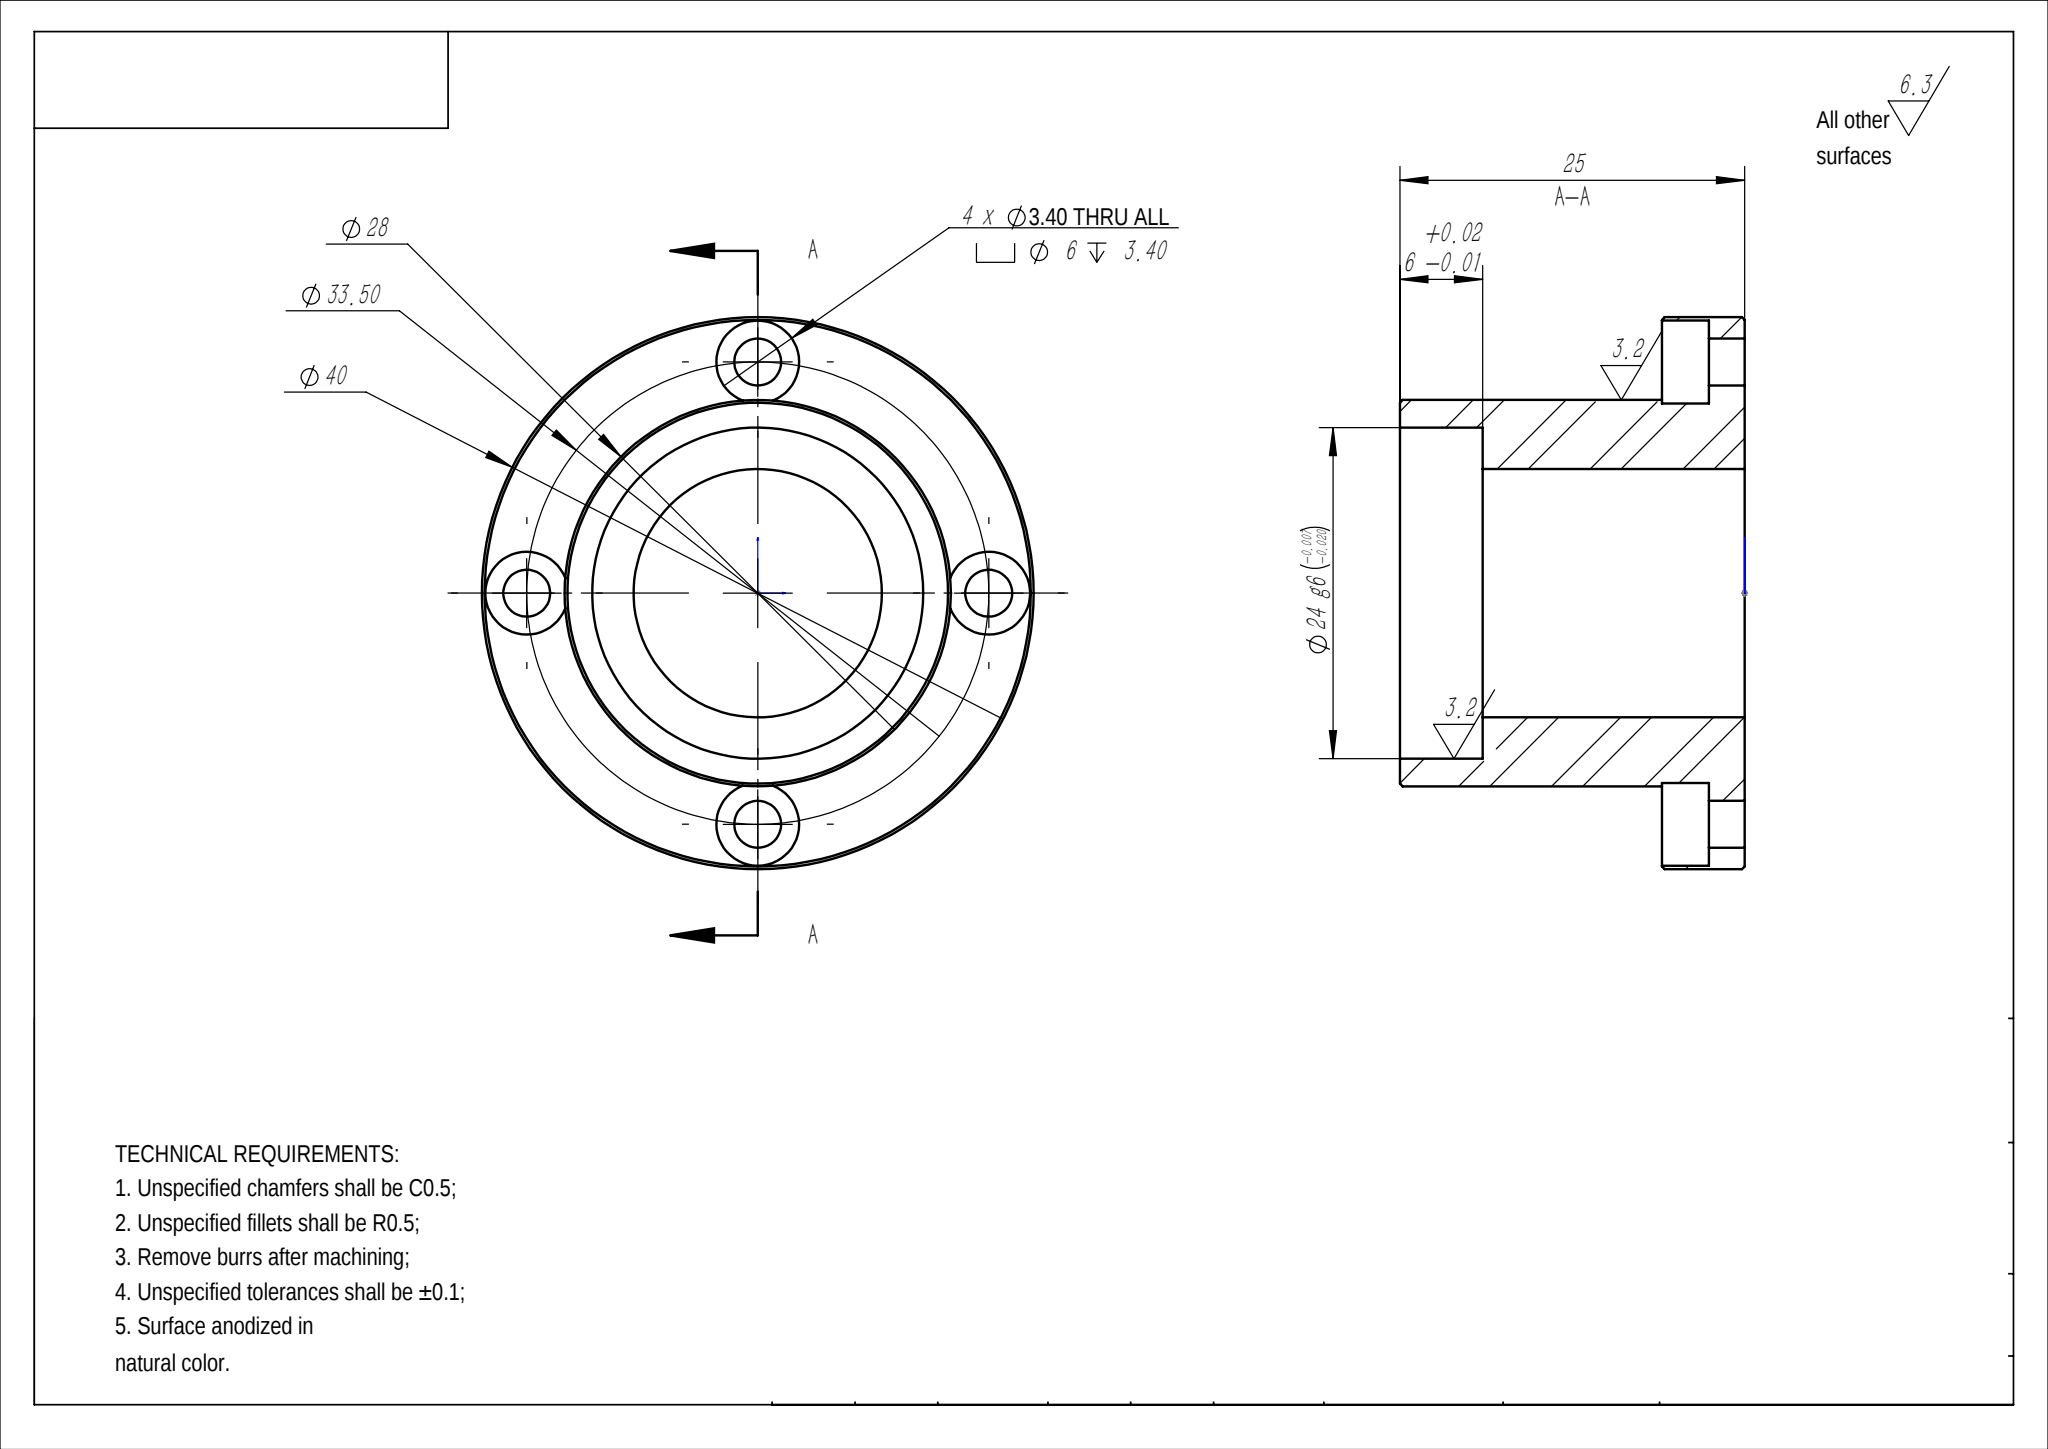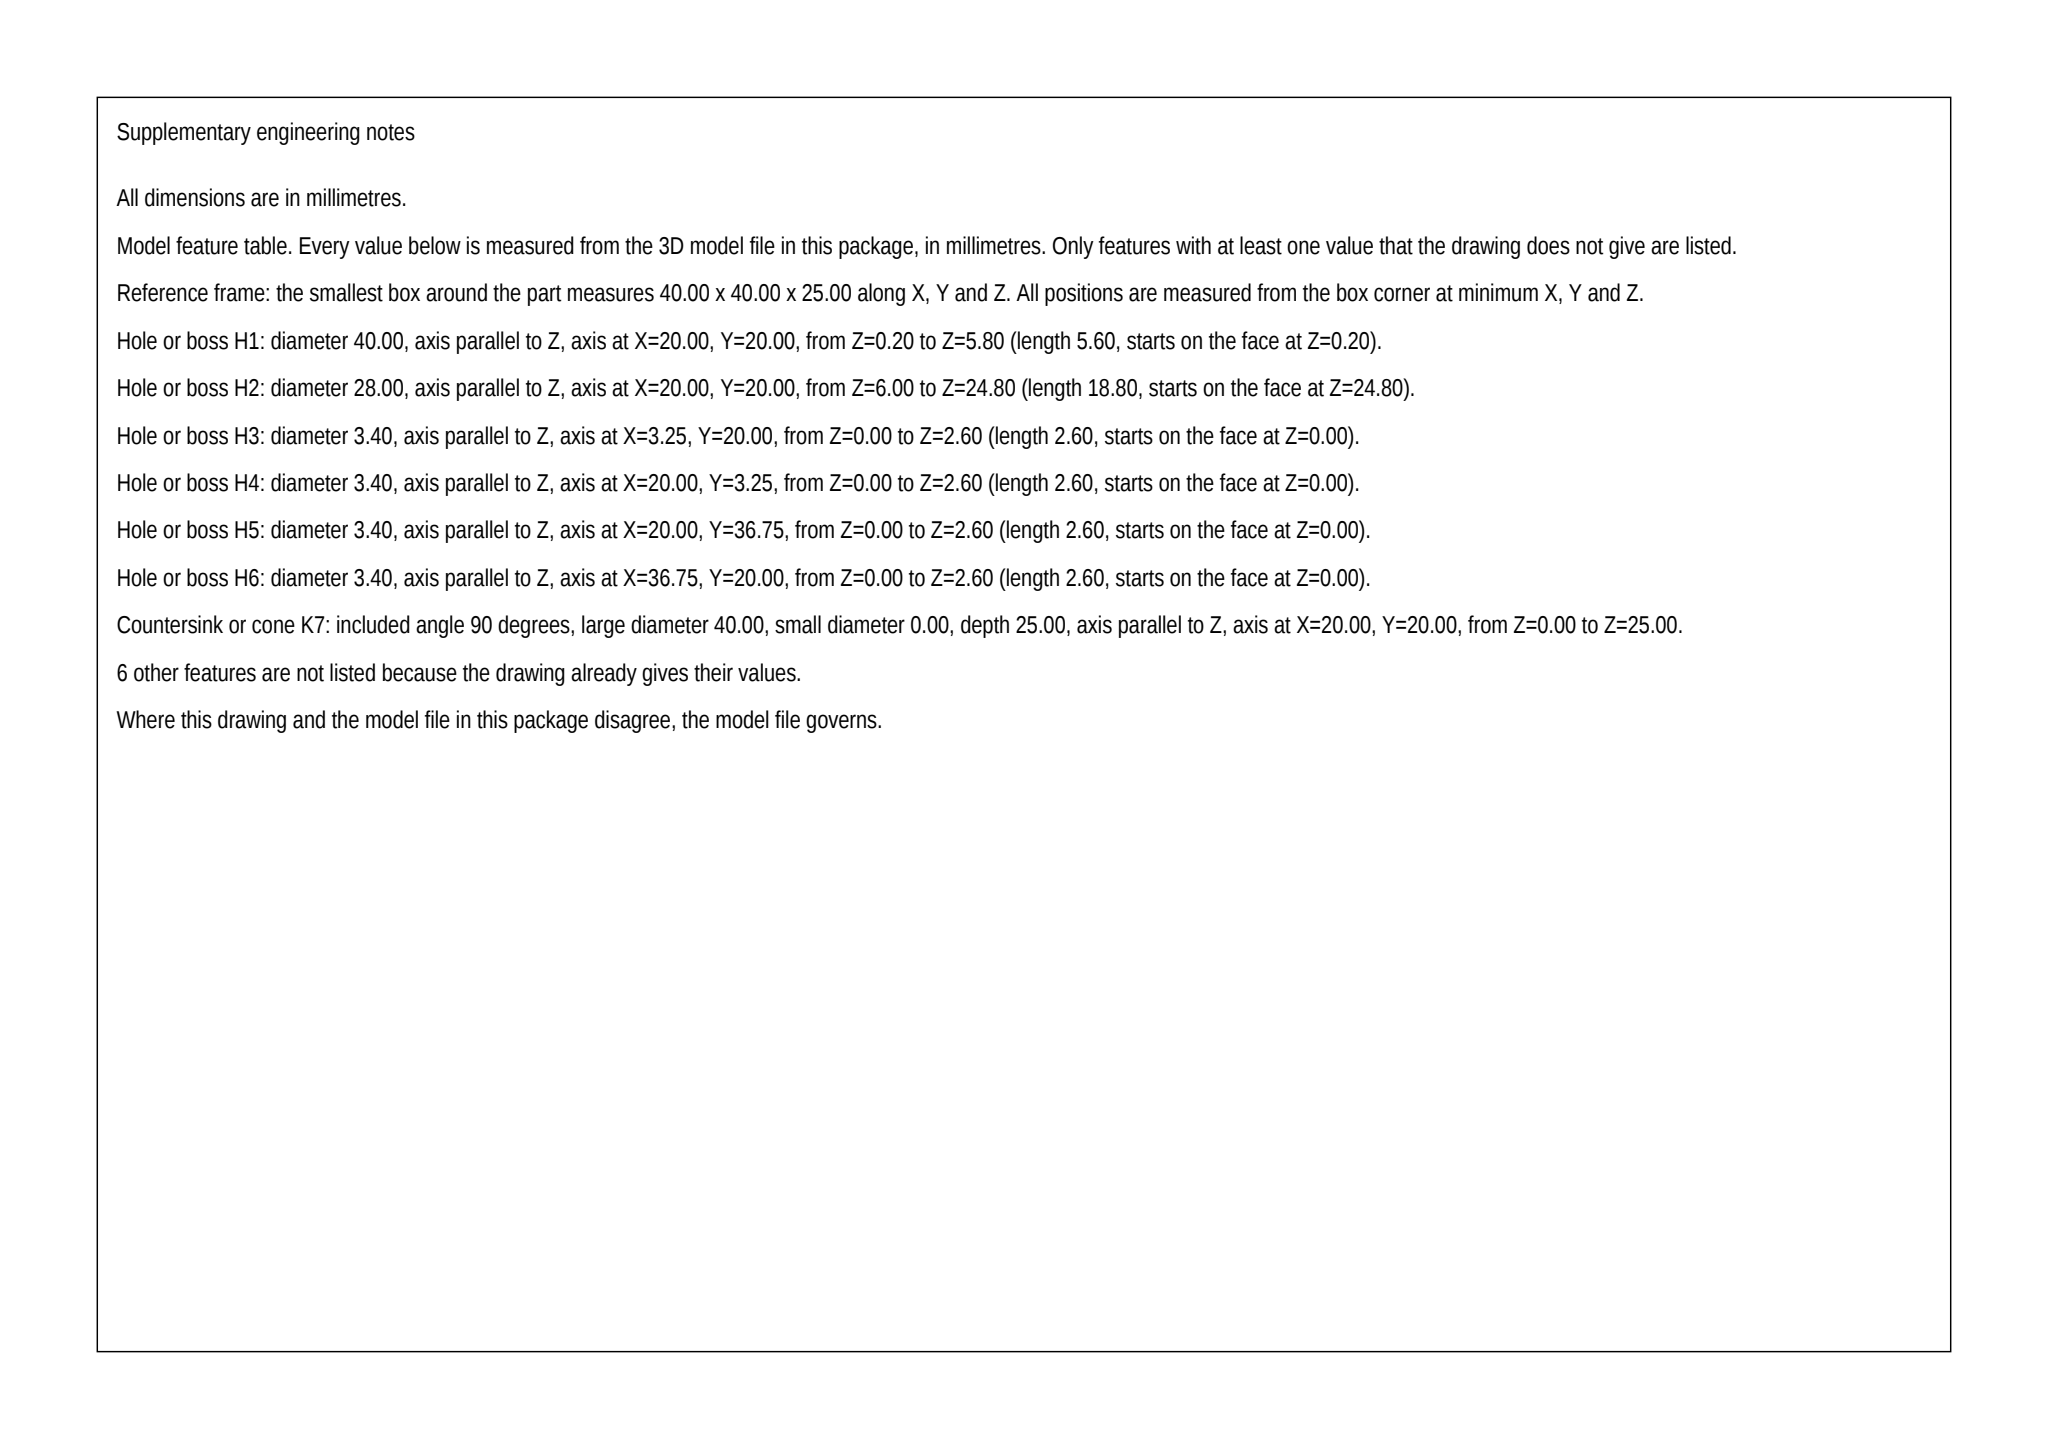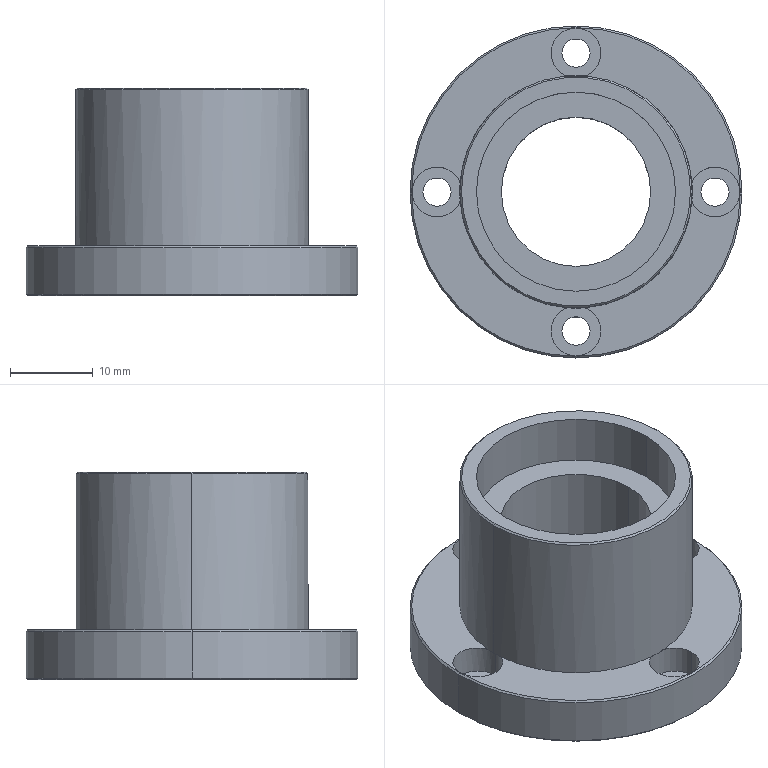Part | SolidWorks | mm | 1 solid | 42 faces | box 40 x 40 x 25 mm | volume 11204 mm3 | cylinder 24 | plane 12 | cone 6 | commonest cylinder face diameters 6 x8 3.4 x8 28 x2 24 x2 18 x2 40 x2
build123d program:
from build123d import *

# Parameters (mm, degrees)
SKETCH1_R                                 = 20
SKETCH1_R_2                               = 9
BOSS_EXTRUDE1_DEPTH                       = 25
SKETCH3_R                                 = 12
CUT_EXTRUDE1_DEPTH                        = 6
CUT_EXTRUDE2_START                        = -19
SKETCH4_R                                 = 20
SKETCH4_R_2                               = 14
CUT_EXTRUDE2_DEPTH                        = 19
HOLE_SIZE_ACCORDING_TO_HEXAGON_SO_2_COUNT = 2
HOLE_SIZE_ACCORDING_TO_HEXAGON_SO_2_PITCH = 23.688
HOLE_SIZE_ACCORDING_TO_HEXAGON_SO_3_COUNT = 2
HOLE_SIZE_ACCORDING_TO_HEXAGON_SO_3_PITCH = 33.5
HOLE_SIZE_ACCORDING_TO_HEXAGON_SO_4_COUNT = 2
HOLE_SIZE_ACCORDING_TO_HEXAGON_SO_4_PITCH = 23.688
HOLE_SIZE_ACCORDING_TO_HEXAGON_SO_5_COUNT = 2
HOLE_SIZE_ACCORDING_TO_HEXAGON_SO_5_PITCH = 16.75
CHAMFER1_SIZE                             = 0.2


with BuildPart() as part:
    # Sketch1 → Boss-Extrude1 (new body)
    with BuildSketch(Plane.XY):
        Circle(SKETCH1_R)
        Circle(SKETCH1_R_2, mode=Mode.SUBTRACT)
    extrude(amount=BOSS_EXTRUDE1_DEPTH)

    # Sketch3 → Cut-Extrude1 (cut)
    with BuildSketch(Plane.XY.offset(25)):
        Circle(SKETCH3_R)
    extrude(amount=-CUT_EXTRUDE1_DEPTH, mode=Mode.SUBTRACT)

    # Sketch4 → Cut-Extrude2 (cut)
    with BuildSketch(Plane.XY.offset(25).offset(CUT_EXTRUDE2_START)):
        Circle(SKETCH4_R)
        Circle(SKETCH4_R_2, mode=Mode.SUBTRACT)
    extrude(amount=CUT_EXTRUDE2_DEPTH, mode=Mode.SUBTRACT)

    # Sketch5 → Hole Size _ according to_ Hexagon Socket (revolve, cut)
    with BuildSketch(Plane(origin=(0, 16.75, 6), x_dir=(0, -1, 0), z_dir=(1, 0, 0))):
        Polygon((0, 0), (0, 6), (1.7, 6), (1.7, 3.4), (3, 3.4), (3, 0), align=None)
    hole_size_according_to_hexagon_socket = revolve(axis=Axis((0, 16.75, 12.35), (0, 0, -1)), mode=Mode.SUBTRACT)

    # Hole Size _ according to_ Hexagon So 2: Hole Size _ according to_ Hexagon Socket ×2
    with Locations(*[Vector(0.7071, -0.7071, 0) * (i * HOLE_SIZE_ACCORDING_TO_HEXAGON_SO_2_PITCH) for i in range(1, HOLE_SIZE_ACCORDING_TO_HEXAGON_SO_2_COUNT)]):
        add(hole_size_according_to_hexagon_socket, mode=Mode.SUBTRACT)

    # Hole Size _ according to_ Hexagon So 3: Hole Size _ according to_ Hexagon Socket ×2
    with Locations(*[(0, -i * HOLE_SIZE_ACCORDING_TO_HEXAGON_SO_3_PITCH, 0) for i in range(1, HOLE_SIZE_ACCORDING_TO_HEXAGON_SO_3_COUNT)]):
        add(hole_size_according_to_hexagon_socket, mode=Mode.SUBTRACT)

    # Hole Size _ according to_ Hexagon So 4: Hole Size _ according to_ Hexagon Socket ×2
    with Locations(*[Vector(-0.7071, -0.7071, 0) * (i * HOLE_SIZE_ACCORDING_TO_HEXAGON_SO_4_PITCH) for i in range(1, HOLE_SIZE_ACCORDING_TO_HEXAGON_SO_4_COUNT)]):
        add(hole_size_according_to_hexagon_socket, mode=Mode.SUBTRACT)

    # Hole Size _ according to_ Hexagon So 5: Hole Size _ according to_ Hexagon Socket ×2
    with Locations(*[(0, -i * HOLE_SIZE_ACCORDING_TO_HEXAGON_SO_5_PITCH, 0) for i in range(1, HOLE_SIZE_ACCORDING_TO_HEXAGON_SO_5_COUNT)]):
        add(hole_size_according_to_hexagon_socket, mode=Mode.SUBTRACT)

    # Chamfer1
    chamfer1_edges = [part.edges().sort_by_distance(p)[0] for p in [
        (-20, 0, 6),
        (-14, 0, 25),
        (-20, 0, 0),
    ]]
    chamfer(chamfer1_edges, length=CHAMFER1_SIZE)


solid = part.part